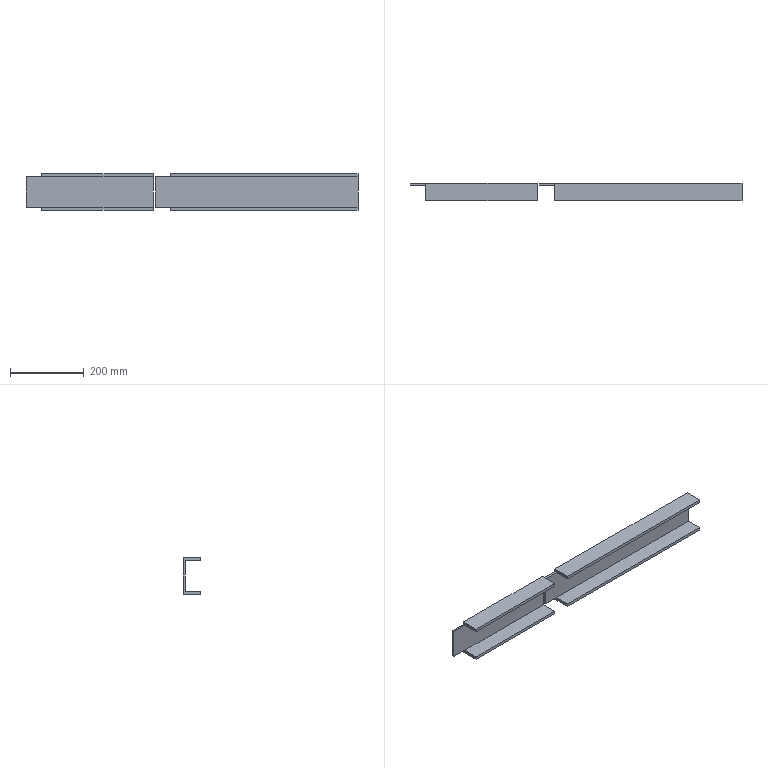Component | NX | CHUNSHUIJINCAO_CAOGANG3 | 2 solids | 28 faces | volume 1053591 mm3 | plane 28